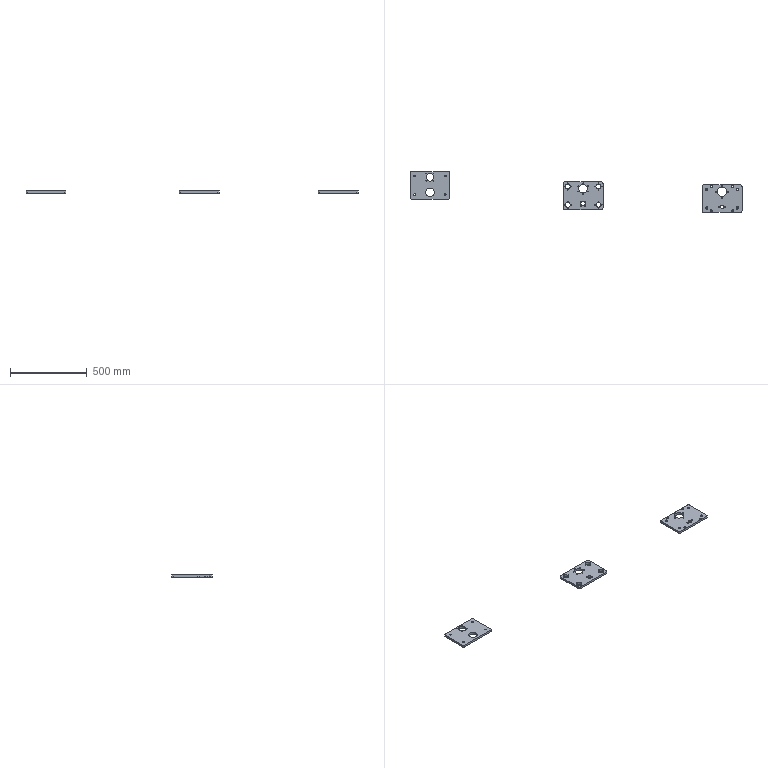CAM job | Mastercam | mm | 12 operations | part box 2728.38 x 1148.46 x 14
1. Facing | 24 - 63 平铣刀
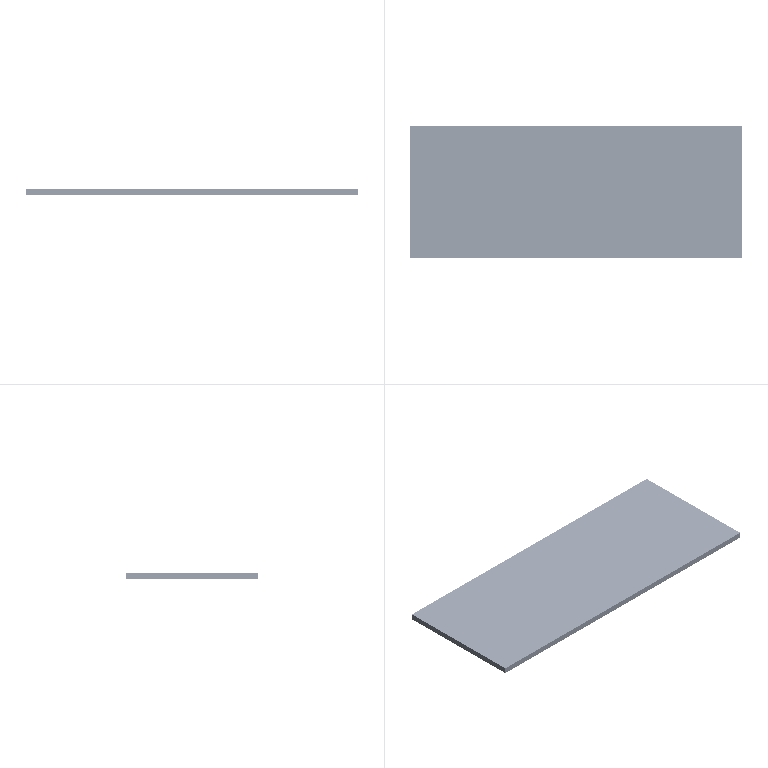2. Contour (Ramp) | 12 - 12 平铣刀
3. 2D High Speed (2D Dynamic Mill) | 12 - 12 平铣刀
4. Contour (2D) | 13 - 12 平铣刀
5. Contour (2D) | 13 - 12 平铣刀
6. Contour (2D) | 13 - 12 平铣刀
7. Drill/Counterbore | 7 - 6 倒角刀
8. Peck Drill | 1 - 10.5 钻头
9. Peck Drill | 2 - 4.3 钻头
10. Contour (2D chamfer) | 7 - 6 倒角刀
11. Contour (2D chamfer) | 7 - 6 倒角刀
12. Tap | 3 - M5 x 0.8 右牙